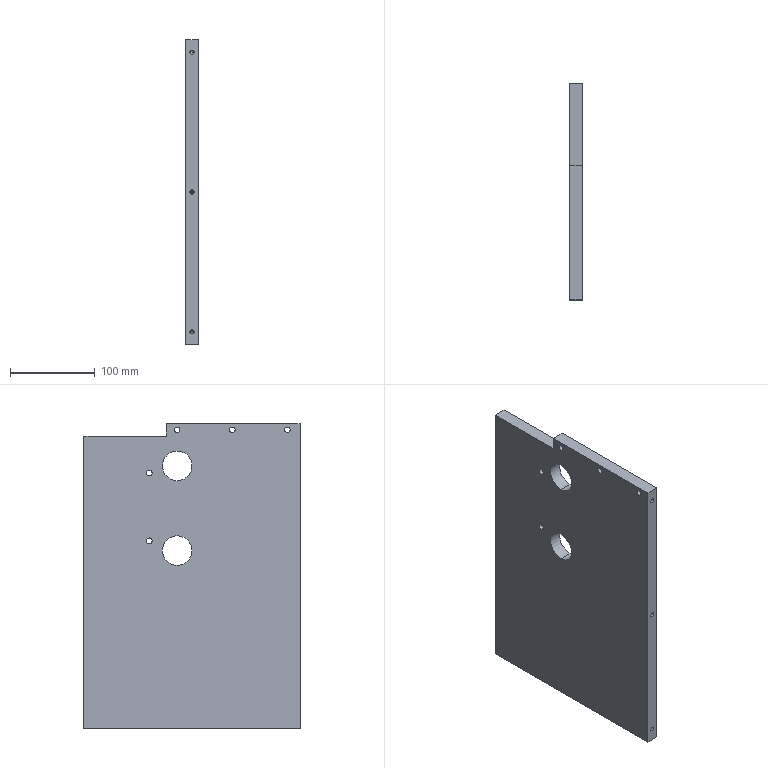Component | SolidWorks | SideFixingPlate2-1 | 1 solid | 69 faces | box 15 x 255 x 360 mm | volume 1318417 mm3 | cylinder 38 | cone 20 | plane 11 | commonest cylinder face diameters 5 x12 6.8 x10 11 x6 6.6 x6 35 x4 | material 1060 Alloy
build123d program:
from build123d import *

# Parameters (mm, degrees)
SKETCH1_W                                          = 360
SKETCH1_H                                          = 255
BOSS_EXTRUDE1_DEPTH                                = 15
HOLE_SIZE_ACCORDING_TO_TYPE_OF_HEXAGON_D           = 6.6
HOLE_SIZE_ACCORDING_TO_TYPE_OF_HEXAGON_CBORE_D     = 11
HOLE_SIZE_ACCORDING_TO_TYPE_OF_HEXAGON_CBORE_DEPTH = 6.8
SKETCH7_W                                          = 15
SKETCH7_H                                          = 97
CUT_EXTRUDE1_DEPTH                                 = 383.206
M8_TAPPED_HOLE1_D                                  = 6.8
M8_TAPPED_HOLE2_D                                  = 6.8
M8_TAPPED_HOLE2_DEPTH                              = 19.75
M8_TAPPED_HOLE2_TIP                                = 2.043
SKETCH12_R                                         = 17.5
CUT_EXTRUDE2_DEPTH                                 = 383.206
M6_TAPPED_HOLE1_D                                  = 5
M6_TAPPED_HOLE1_DEPTH                              = 15
M6_TAPPED_HOLE1_TIP                                = 1.502
M6_TAPPED_HOLE2_D                                  = 5
M6_TAPPED_HOLE2_DEPTH                              = 15
M6_TAPPED_HOLE2_TIP                                = 1.502


with BuildPart() as part:
    # Sketch1 → Boss-Extrude1 (new body)
    with BuildSketch(Plane.XY):
        with Locations((180, 0)):
            Rectangle(SKETCH1_W, SKETCH1_H)
    extrude(amount=BOSS_EXTRUDE1_DEPTH)

    # Hole Size _according to_ type of Hexagon (through all)
    with Locations(Plane.XY.offset(15)):
        with Locations((7.5, 17.5), (7.5, -47.5), (7.5, -112.5)):
            CounterBoreHole(HOLE_SIZE_ACCORDING_TO_TYPE_OF_HEXAGON_D / 2, HOLE_SIZE_ACCORDING_TO_TYPE_OF_HEXAGON_CBORE_D / 2, HOLE_SIZE_ACCORDING_TO_TYPE_OF_HEXAGON_CBORE_DEPTH)

    # Sketch7 → Cut-Extrude1 (cut, through all)
    with BuildSketch(Plane.XY.offset(15)):
        with Locations((7.5, 79)):
            Rectangle(SKETCH7_W, SKETCH7_H)
    extrude(amount=-CUT_EXTRUDE1_DEPTH, mode=Mode.SUBTRACT)

    # M8 Tapped Hole1 (through all)
    with Locations(Plane.XY.offset(15)):
        with Locations((58.5, 50.5), (138.5, 50.5)):
            Hole(M8_TAPPED_HOLE1_D / 2)

    # M8 Tapped Hole2
    with Locations(Plane(origin=(0, 127.5, 0), x_dir=(1, 0, 0), z_dir=(0, 1, 0))):
        with Locations((335, -7.5), (185, -7.5), (85, -7.5)):
            Hole(M8_TAPPED_HOLE2_D / 2, depth=M8_TAPPED_HOLE2_DEPTH)
            with Locations((0, 0, -(M8_TAPPED_HOLE2_DEPTH + M8_TAPPED_HOLE2_TIP / 2))):  # 118° drill point
                Cone(0, M8_TAPPED_HOLE2_D / 2, M8_TAPPED_HOLE2_TIP, mode=Mode.SUBTRACT)

    # Sketch12 → Cut-Extrude2 (cut, through all)
    with BuildSketch(Plane.XY.offset(15)):
        with Locations((50, 17.5)):
            Circle(SKETCH12_R)
        with Locations((150, 17.5)):
            Circle(SKETCH12_R)
    extrude(amount=-CUT_EXTRUDE2_DEPTH, mode=Mode.SUBTRACT)

    # M6 Tapped Hole1
    with Locations(Plane(origin=(360, 0, 0), x_dir=(0, 0, -1), z_dir=(1, 0, 0))):
        with Locations((-7.5, -112), (-7.5, 0), (-7.5, 112)):
            Hole(M6_TAPPED_HOLE1_D / 2, depth=M6_TAPPED_HOLE1_DEPTH)
            with Locations((0, 0, -(M6_TAPPED_HOLE1_DEPTH + M6_TAPPED_HOLE1_TIP / 2))):  # 118° drill point
                Cone(0, M6_TAPPED_HOLE1_D / 2, M6_TAPPED_HOLE1_TIP, mode=Mode.SUBTRACT)

    # M6 Tapped Hole2
    with Locations(Plane(origin=(0, -127.5, 0), x_dir=(-1, 0, 0), z_dir=(0, -1, 0))):
        with Locations((-345, -7.5), (-180, -7.5), (-15, -7.5)):
            Hole(M6_TAPPED_HOLE2_D / 2, depth=M6_TAPPED_HOLE2_DEPTH)
            with Locations((0, 0, -(M6_TAPPED_HOLE2_DEPTH + M6_TAPPED_HOLE2_TIP / 2))):  # 118° drill point
                Cone(0, M6_TAPPED_HOLE2_D / 2, M6_TAPPED_HOLE2_TIP, mode=Mode.SUBTRACT)


solid = part.part

# Placed as in the assembly
solid = solid.moved(Location((35.334, 87.764, 197.5), (0, 90, 0)))